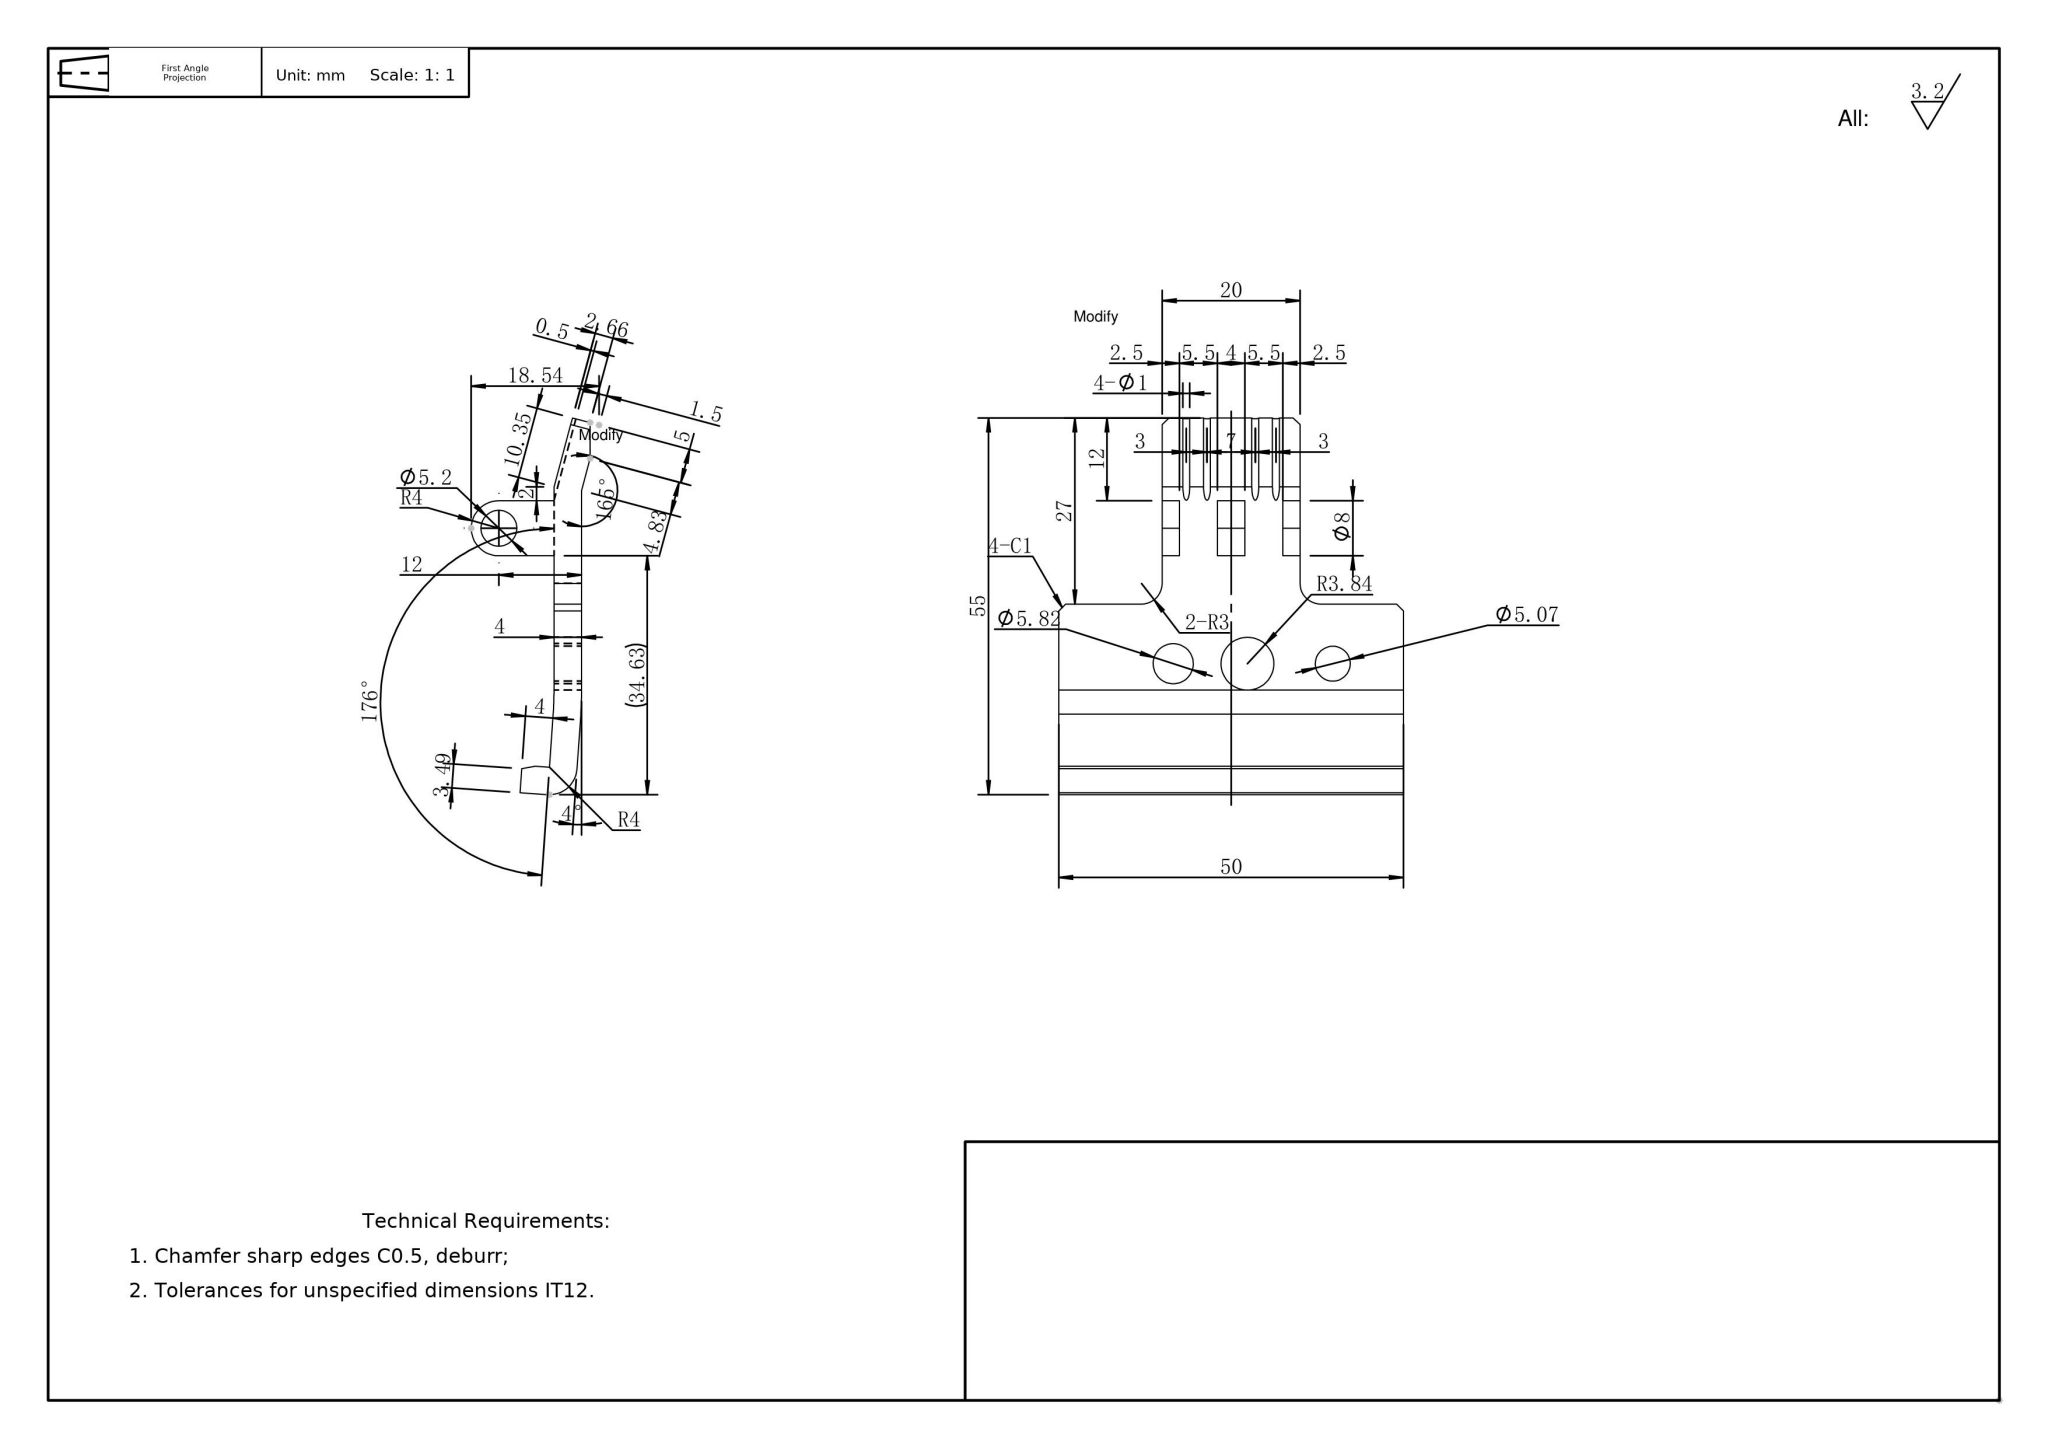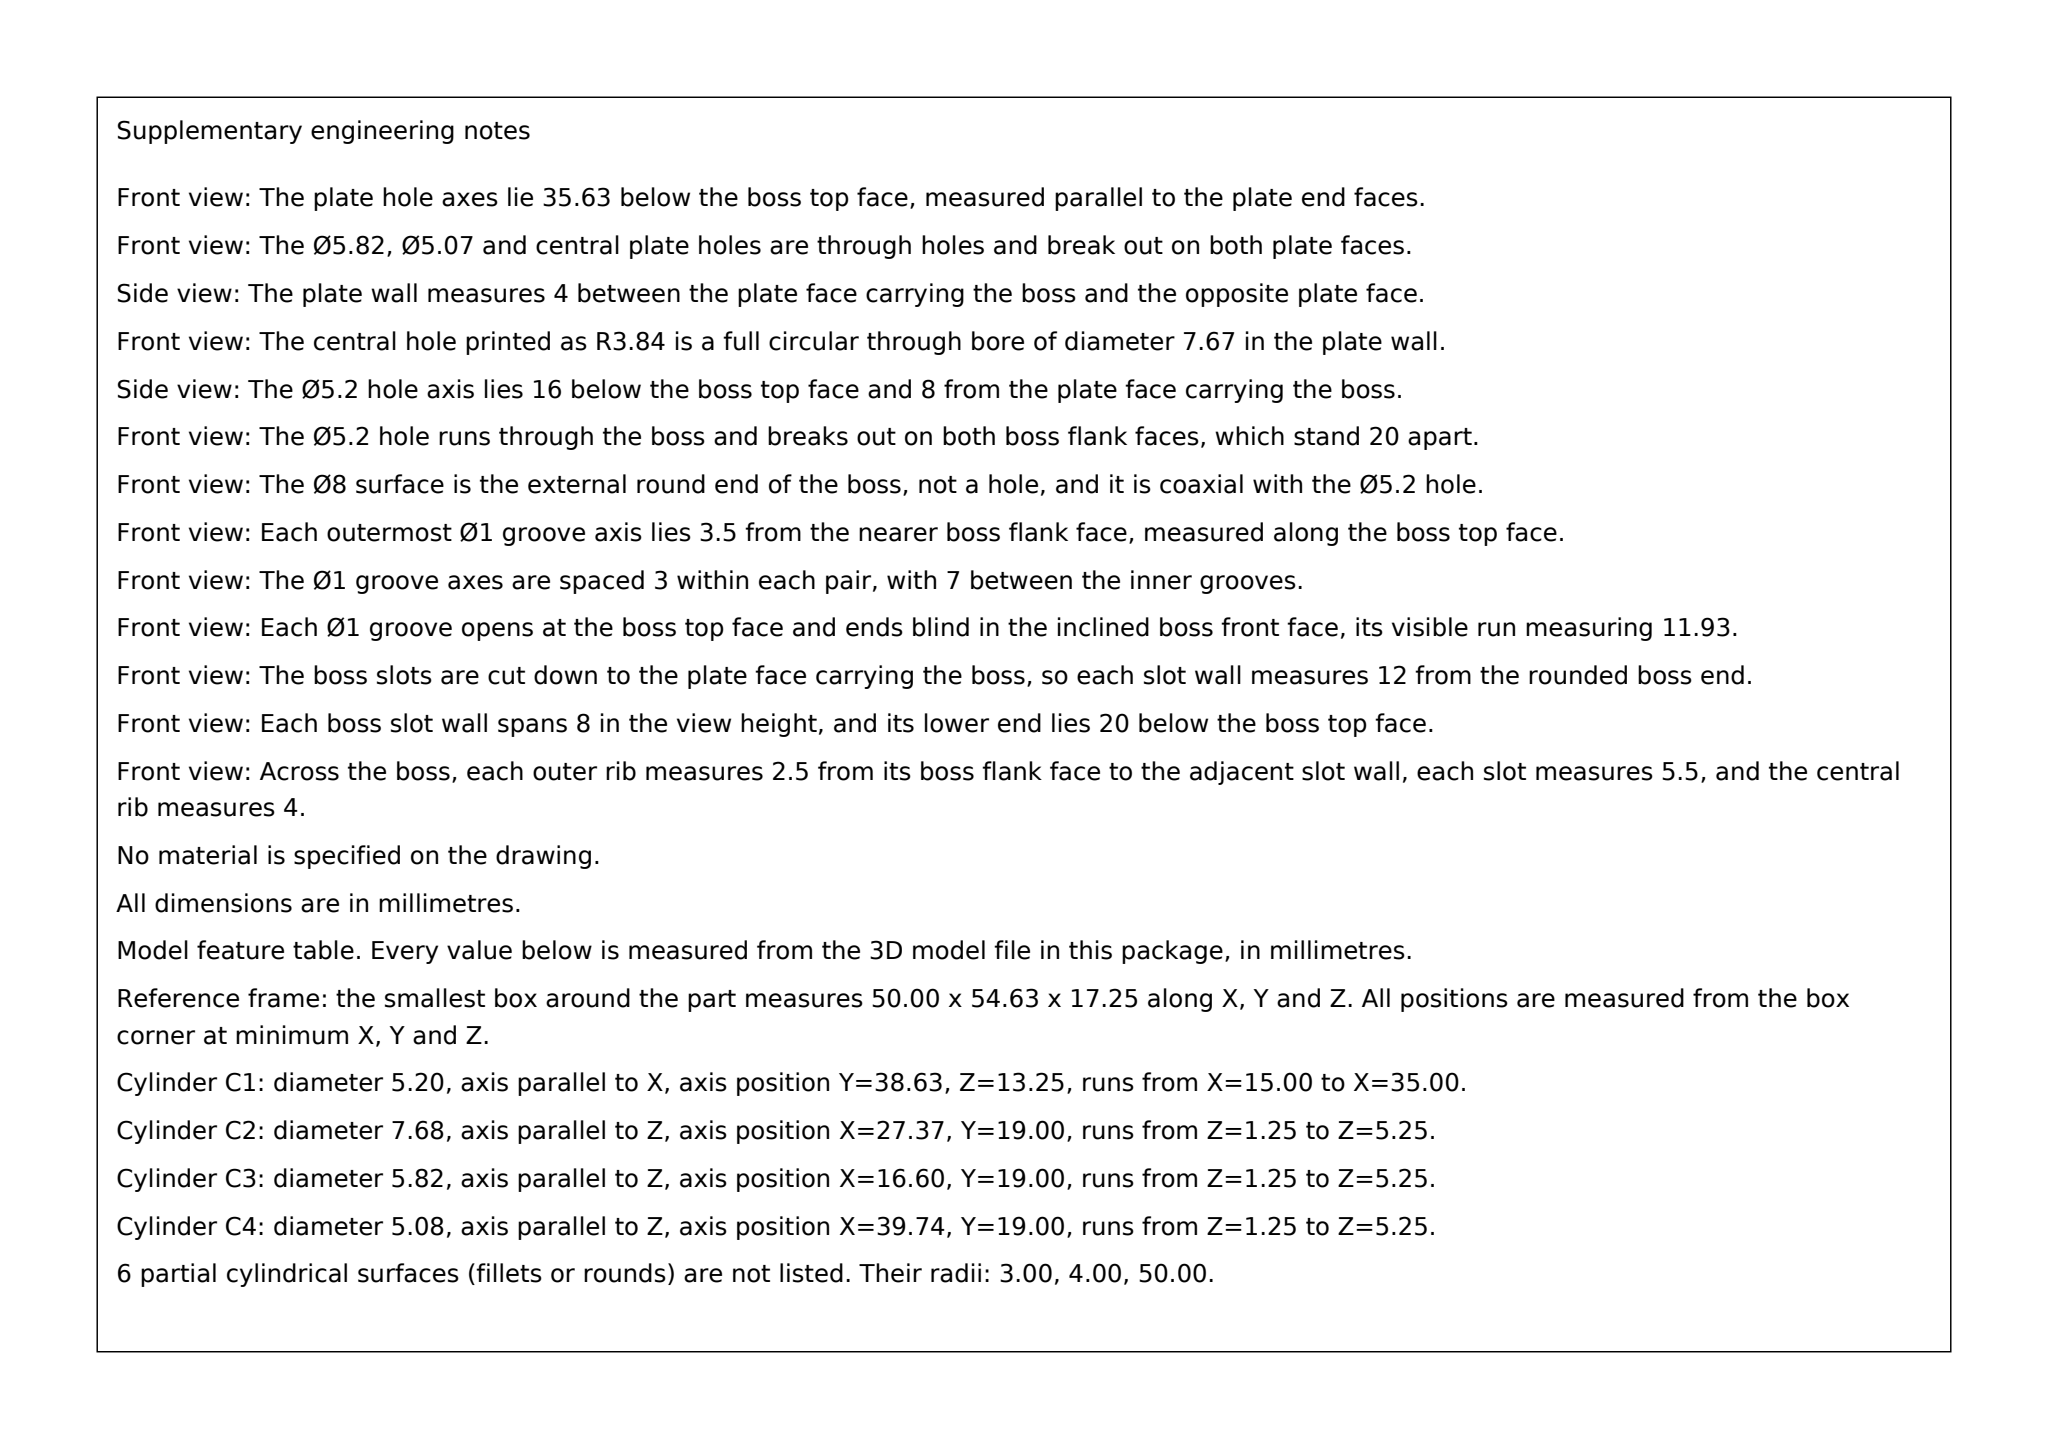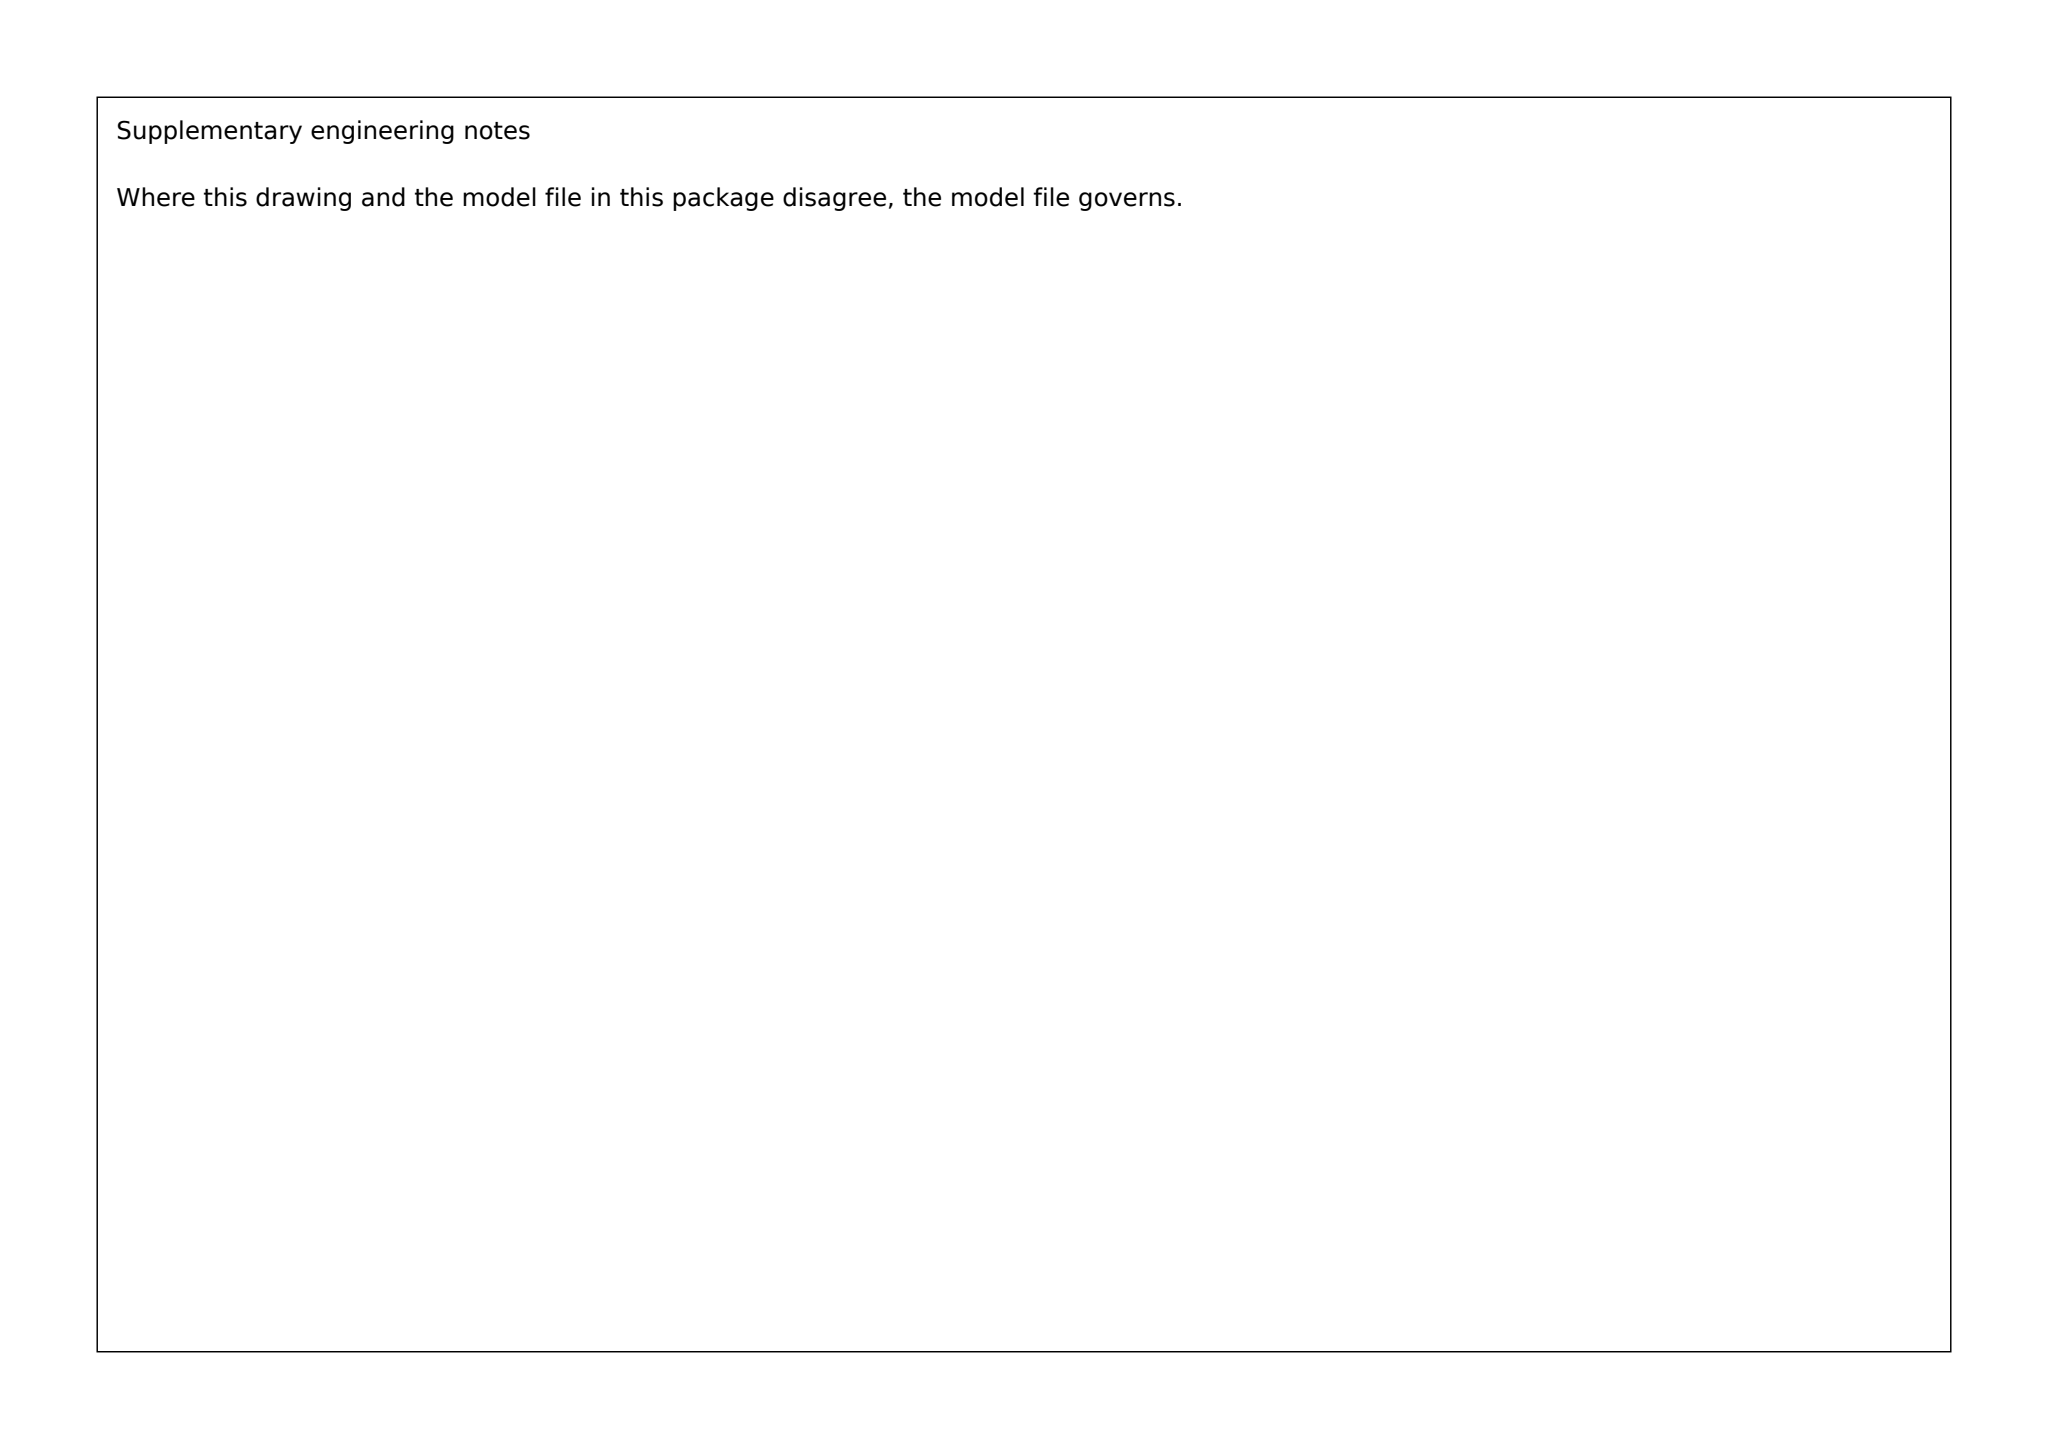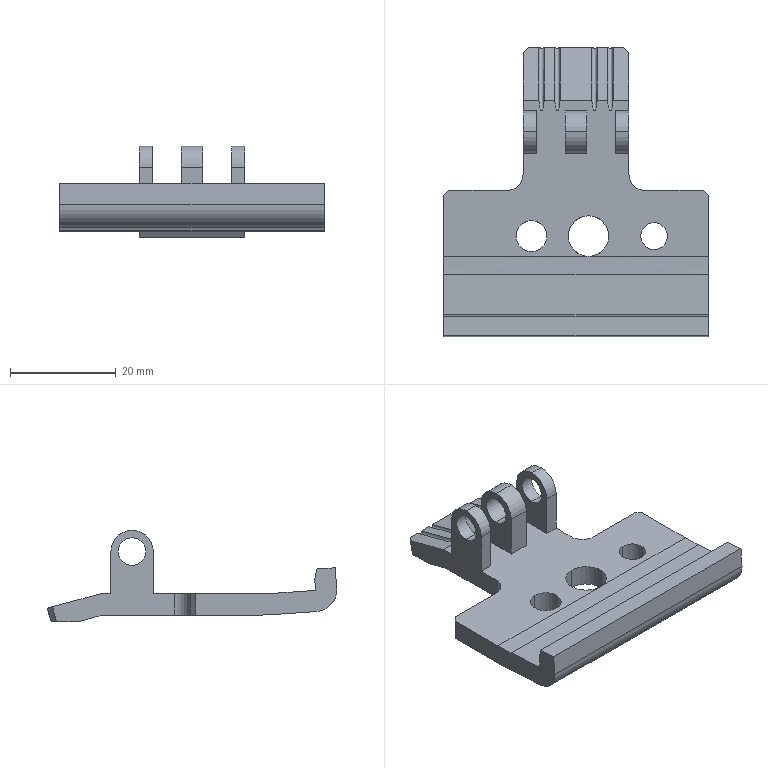Part | SolidWorks | mm | 1 solid | 63 faces | box 50 x 54.63 x 17.25 mm | volume 8472 mm3 | plane 36 | cylinder 27 | commonest cylinder face diameters 8 x7 5.2 x6 1 x4 5.071 x2 5.824 x2 7.67 x2 100 x2 6 x2
Drawing notes:
FRONT VIEW: Ø5.82, Ø7.67 & Ø5.07 CL 16.6, 27.37 & 39.74 FROM LH EDGE | from the solid: cyl dia 5.824 @x=16.6, dia 7.67 @x=27.37, dia 5.071 @x=39.74 (z-axis holes); bbox x 0-50
Ø5.82/Ø7.67/Ø5.07 CL 19 ABV BOT EDGE, THRU 4 | from the solid: all three z-axis holes at y=19.0, length 4 = plate thk; bbox y 0-54.631
2-R3 (Ø6) CL 12 & 38 FROM LH EDGE, 24 BELOW TOP EDGE | from the solid: dia 6.0 z-axis cyls at (12.0,30.63) and (38.0,30.63); 54.631-30.63=24
4-Ø1 VERT HOLES DP 11.94 FROM TOP EDGE (END 12 BELOW TOP) | from the solid: dia 1.0 y-axis cyls, length 11.94, top face y=54.631, y-plane 42.63
Ø8/Ø5.2 CURL CL 16 BELOW TOP EDGE; SEGS 4 x 2.5 + 2 x 4 LG | from the solid: dia 8.0 & 5.2 x-axis cyls at y=38.63, z=13.25, lengths 2.5 (x4) and 4 (x2); 54.631-38.63=16
Ø8 RELIEF ALONG BOT EDGE: CL 4 ABV BOT EDGE, 50 LG FULL WIDTH | from the solid: dia 8.0 x-axis cyl at y=4.0, z=5.91, length 50 = full part width
MATL THK 4 THRU-OUT | from the solid: z-planes 1.25 & 5.25; Ø100 form surfaces offset z 51.25/55.25 = 4 apart
TABS: 4 x 2.5 WIDE + 2 x 4 WIDE WITHIN 20 OVERALL | from the solid: Ø5.2/Ø8 x-axis cyl lengths 2.5 (count 4) & 4 (count 2); x-planes 15 & 35
LARGE FORMED CURVE: R50 (Ø100), 176° INCL, 50 WIDE | from the solid: cylinders dia 100.0 axis x, len 50.0, at y15.04/z51.25 and y15.18/z55.25
Ø8 GROOVE x50 LG: AXIS 4 ABV BOT EDGE, 5.91 FROM REAR FACE | from the solid: cylinder [8.0,'x',[null,4.0,5.91],50.0,1]; bbox from min corner z=0 rear face
CURL TABS 2.5 W @15 & @32.5, 4 W @23 FROM LH EDGE; 5.5 GAPS | from the solid: x-planes 15.0/17.5/23.0/27.0/32.5/35.0; dia5.2&8 x-cyls len 2.5 (x4 faces) + len 4 (x2 faces)
4-Ø1 HOLE AXES 6.45 FROM REAR FACE, DP 11.94 FROM TOP EDGE | from the solid: cylinders dia 1.0 axis y at x18.5/21.5/28.5/31.5, z=6.45, len 11.94
13. Ø8/Ø5.2 CURL AXIS 13.25 FROM REAR FACE (DATUM = REAR FLAT FACE, Z0) | from the solid: cylinders dia 8.0 and 5.2 about x-axis at pos_other_axes [null, 38.63, 13.25]
14. OVERALL FORMED DEPTH 17.25 FROM REAR FACE TO FOREMOST FORMED SURFACE | from the solid: bbox_xyz z extent = 17.249 with rear face plane z=0.0